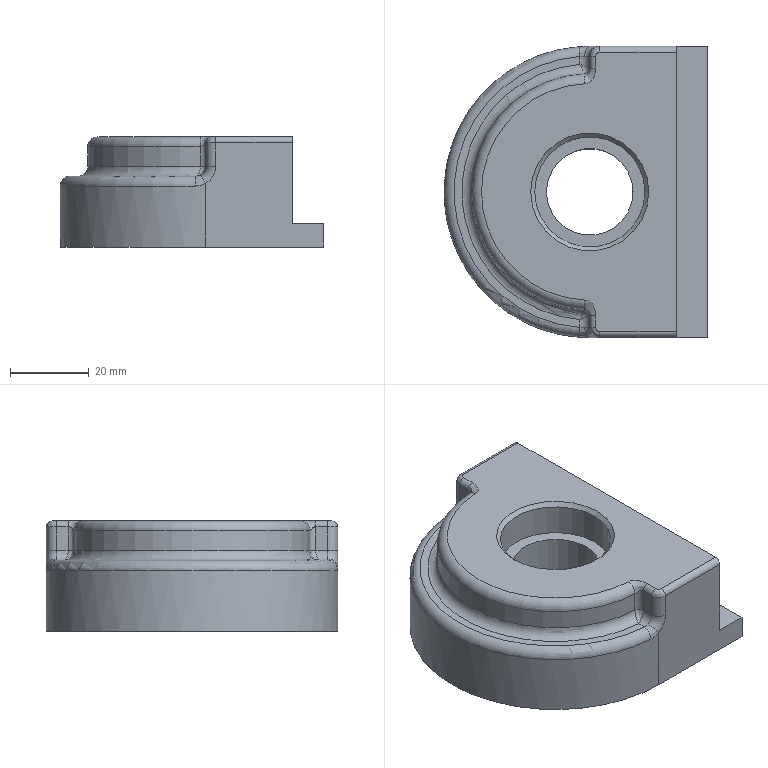Component | NX | 3 | 1 solid | 43 faces | volume 87546 mm3 | cylinder 16 | plane 11 | spline 8 | torus 5 | cone 3 | commonest cylinder face diameters 3 x6 5 x4 8 x2 74 x1 60 x1 28 x1 22 x1